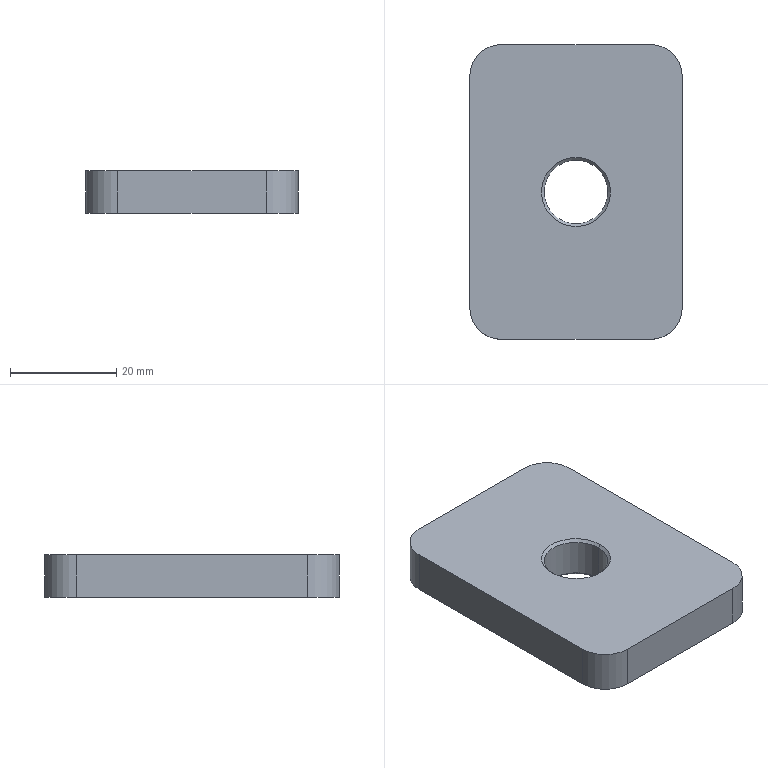Component | SolidWorks | 01-01Chassis-1_01-01-03ChassisWeldment3-1 | 1 solid | 16 faces | box 40 x 55.5 x 8 mm | volume 16598 mm3 | cylinder 6 | plane 6 | cone 4 | commonest cylinder face diameters 12 x6 | material Q235
STEP:
#1=COLOUR_RGB('',0.7922,0.8196,0.9333);
#2=FILL_AREA_STYLE_COLOUR('',#1);
#3=FILL_AREA_STYLE('',(#2));
#4=SURFACE_STYLE_FILL_AREA(#3);
#5=SURFACE_SIDE_STYLE('',(#4));
#6=SURFACE_STYLE_USAGE(.BOTH.,#5);
#7=PRESENTATION_STYLE_ASSIGNMENT((#6));
#8=CARTESIAN_POINT('',(11.575,-2.096,17.815));
#9=VERTEX_POINT('',#8);
#10=CARTESIAN_POINT('',(12.047,-2.096,17.815));
#11=VERTEX_POINT('',#10);
#12=CARTESIAN_POINT('',(11.811,-2.096,17.815));
#13=DIRECTION('',(0.,-0.,1.));
#14=DIRECTION('',(-1.,0.,0.));
#15=AXIS2_PLACEMENT_3D('',#12,#13,#14);
#16=CIRCLE('',#15,0.2362);
#17=EDGE_CURVE('',#9,#11,#16,.T.);
#18=ORIENTED_EDGE('',*,*,#17,.F.);
#19=CARTESIAN_POINT('',(11.555,-2.096,17.835));
#20=VERTEX_POINT('',#19);
#21=CARTESIAN_POINT('',(11.575,-2.096,17.815));
#22=DIRECTION('',(-0.7071,-0.,0.7071));
#23=VECTOR('',#22,39.37);
#24=LINE('',#21,#23);
#25=EDGE_CURVE('',#9,#20,#24,.T.);
#26=ORIENTED_EDGE('',*,*,#25,.T.);
#27=CARTESIAN_POINT('',(12.067,-2.096,17.835));
#28=VERTEX_POINT('',#27);
#29=CARTESIAN_POINT('',(11.811,-2.096,17.835));
#30=DIRECTION('',(-0.,0.,-1.));
#31=DIRECTION('',(-1.,0.,0.));
#32=AXIS2_PLACEMENT_3D('',#29,#30,#31);
#33=CIRCLE('',#32,0.2559);
#34=EDGE_CURVE('',#28,#20,#33,.T.);
#35=ORIENTED_EDGE('',*,*,#34,.F.);
#36=CARTESIAN_POINT('',(12.047,-2.096,17.815));
#37=DIRECTION('',(0.7071,-0.,0.7071));
#38=VECTOR('',#37,39.37);
#39=LINE('',#36,#38);
#40=EDGE_CURVE('',#11,#28,#39,.T.);
#41=ORIENTED_EDGE('',*,*,#40,.F.);
#42=EDGE_LOOP('',(#18,#26,#35,#41));
#43=FACE_OUTER_BOUND('',#42,.T.);
#44=CARTESIAN_POINT('',(11.811,-2.096,17.815));
#45=DIRECTION('',(0.,-0.,1.));
#46=DIRECTION('',(1.,0.,0.));
#47=AXIS2_PLACEMENT_3D('',#44,#45,#46);
#48=CONICAL_SURFACE('',#47,0.2362,0.7854);
#49=ADVANCED_FACE('',(#43),#48,.F.);
#50=CARTESIAN_POINT('',(12.047,-2.096,17.539));
#51=VERTEX_POINT('',#50);
#52=CARTESIAN_POINT('',(11.575,-2.096,17.539));
#53=VERTEX_POINT('',#52);
#54=CARTESIAN_POINT('',(11.811,-2.096,17.539));
#55=DIRECTION('',(-0.,0.,-1.));
#56=DIRECTION('',(-1.,0.,0.));
#57=AXIS2_PLACEMENT_3D('',#54,#55,#56);
#58=CIRCLE('',#57,0.2362);
#59=EDGE_CURVE('',#51,#53,#58,.T.);
#60=ORIENTED_EDGE('',*,*,#59,.F.);
#61=CARTESIAN_POINT('',(12.067,-2.096,17.52));
#62=VERTEX_POINT('',#61);
#63=CARTESIAN_POINT('',(12.047,-2.096,17.539));
#64=DIRECTION('',(0.7071,0.,-0.7071));
#65=VECTOR('',#64,39.37);
#66=LINE('',#63,#65);
#67=EDGE_CURVE('',#51,#62,#66,.T.);
#68=ORIENTED_EDGE('',*,*,#67,.T.);
#69=CARTESIAN_POINT('',(11.555,-2.096,17.52));
#70=VERTEX_POINT('',#69);
#71=CARTESIAN_POINT('',(11.811,-2.096,17.52));
#72=DIRECTION('',(0.,-0.,1.));
#73=DIRECTION('',(-1.,0.,0.));
#74=AXIS2_PLACEMENT_3D('',#71,#72,#73);
#75=CIRCLE('',#74,0.2559);
#76=EDGE_CURVE('',#70,#62,#75,.T.);
#77=ORIENTED_EDGE('',*,*,#76,.F.);
#78=CARTESIAN_POINT('',(11.575,-2.096,17.539));
#79=DIRECTION('',(-0.7071,0.,-0.7071));
#80=VECTOR('',#79,39.37);
#81=LINE('',#78,#80);
#82=EDGE_CURVE('',#53,#70,#81,.T.);
#83=ORIENTED_EDGE('',*,*,#82,.F.);
#84=EDGE_LOOP('',(#60,#68,#77,#83));
#85=FACE_OUTER_BOUND('',#84,.T.);
#86=CARTESIAN_POINT('',(11.811,-2.096,17.539));
#87=DIRECTION('',(-0.,0.,-1.));
#88=DIRECTION('',(-1.,0.,0.));
#89=AXIS2_PLACEMENT_3D('',#86,#87,#88);
#90=CONICAL_SURFACE('',#89,0.2362,0.7854);
#91=ADVANCED_FACE('',(#85),#90,.F.);
#92=ORIENTED_EDGE('',*,*,#59,.T.);
#93=CARTESIAN_POINT('',(11.575,-2.096,17.835));
#94=DIRECTION('',(0.,-0.,1.));
#95=VECTOR('',#94,39.37);
#96=LINE('',#93,#95);
#97=EDGE_CURVE('',#53,#9,#96,.T.);
#98=ORIENTED_EDGE('',*,*,#97,.T.);
#99=ORIENTED_EDGE('',*,*,#17,.T.);
#100=CARTESIAN_POINT('',(12.047,-2.096,17.835));
#101=DIRECTION('',(0.,-0.,1.));
#102=VECTOR('',#101,39.37);
#103=LINE('',#100,#102);
#104=EDGE_CURVE('',#51,#11,#103,.T.);
#105=ORIENTED_EDGE('',*,*,#104,.F.);
#106=EDGE_LOOP('',(#92,#98,#99,#105));
#107=FACE_OUTER_BOUND('',#106,.T.);
#108=CARTESIAN_POINT('',(11.811,-2.096,17.835));
#109=DIRECTION('',(0.,-0.,1.));
#110=DIRECTION('',(1.,0.,0.));
#111=AXIS2_PLACEMENT_3D('',#108,#109,#110);
#112=CYLINDRICAL_SURFACE('',#111,0.2362);
#113=ADVANCED_FACE('',(#107),#112,.F.);
#114=ORIENTED_EDGE('',*,*,#34,.T.);
#115=CARTESIAN_POINT('',(11.811,-2.096,17.835));
#116=DIRECTION('',(-0.,0.,-1.));
#117=DIRECTION('',(-1.,0.,0.));
#118=AXIS2_PLACEMENT_3D('',#115,#116,#117);
#119=CIRCLE('',#118,0.2559);
#120=EDGE_CURVE('',#20,#28,#119,.T.);
#121=ORIENTED_EDGE('',*,*,#120,.T.);
#122=EDGE_LOOP('',(#114,#121));
#123=FACE_BOUND('',#122,.T.);
#124=CARTESIAN_POINT('',(12.362,-1.004,17.835));
#125=VERTEX_POINT('',#124);
#126=CARTESIAN_POINT('',(12.598,-1.24,17.835));
#127=VERTEX_POINT('',#126);
#128=CARTESIAN_POINT('',(12.362,-1.24,17.835));
#129=DIRECTION('',(-0.,0.,-1.));
#130=DIRECTION('',(-1.,0.,0.));
#131=AXIS2_PLACEMENT_3D('',#128,#129,#130);
#132=CIRCLE('',#131,0.2362);
#133=EDGE_CURVE('',#125,#127,#132,.T.);
#134=ORIENTED_EDGE('',*,*,#133,.F.);
#135=CARTESIAN_POINT('',(11.26,-1.004,17.835));
#136=VERTEX_POINT('',#135);
#137=CARTESIAN_POINT('',(11.26,-1.004,17.835));
#138=DIRECTION('',(1.,-0.,-0.));
#139=VECTOR('',#138,39.37);
#140=LINE('',#137,#139);
#141=EDGE_CURVE('',#136,#125,#140,.T.);
#142=ORIENTED_EDGE('',*,*,#141,.F.);
#143=CARTESIAN_POINT('',(11.024,-1.24,17.835));
#144=VERTEX_POINT('',#143);
#145=CARTESIAN_POINT('',(11.26,-1.24,17.835));
#146=DIRECTION('',(-0.,0.,-1.));
#147=DIRECTION('',(1.,0.,0.));
#148=AXIS2_PLACEMENT_3D('',#145,#146,#147);
#149=CIRCLE('',#148,0.2362);
#150=EDGE_CURVE('',#144,#136,#149,.T.);
#151=ORIENTED_EDGE('',*,*,#150,.F.);
#152=CARTESIAN_POINT('',(11.024,-2.953,17.835));
#153=VERTEX_POINT('',#152);
#154=CARTESIAN_POINT('',(11.024,-1.24,17.835));
#155=DIRECTION('',(0.,1.,0.));
#156=VECTOR('',#155,39.37);
#157=LINE('',#154,#156);
#158=EDGE_CURVE('',#153,#144,#157,.T.);
#159=ORIENTED_EDGE('',*,*,#158,.F.);
#160=CARTESIAN_POINT('',(11.26,-3.189,17.835));
#161=VERTEX_POINT('',#160);
#162=CARTESIAN_POINT('',(11.26,-2.953,17.835));
#163=DIRECTION('',(-0.,0.,-1.));
#164=DIRECTION('',(1.,0.,0.));
#165=AXIS2_PLACEMENT_3D('',#162,#163,#164);
#166=CIRCLE('',#165,0.2362);
#167=EDGE_CURVE('',#161,#153,#166,.T.);
#168=ORIENTED_EDGE('',*,*,#167,.F.);
#169=CARTESIAN_POINT('',(12.362,-3.189,17.835));
#170=VERTEX_POINT('',#169);
#171=CARTESIAN_POINT('',(11.26,-3.189,17.835));
#172=DIRECTION('',(-1.,0.,0.));
#173=VECTOR('',#172,39.37);
#174=LINE('',#171,#173);
#175=EDGE_CURVE('',#170,#161,#174,.T.);
#176=ORIENTED_EDGE('',*,*,#175,.F.);
#177=CARTESIAN_POINT('',(12.598,-2.953,17.835));
#178=VERTEX_POINT('',#177);
#179=CARTESIAN_POINT('',(12.362,-2.953,17.835));
#180=DIRECTION('',(-0.,0.,-1.));
#181=DIRECTION('',(1.,0.,0.));
#182=AXIS2_PLACEMENT_3D('',#179,#180,#181);
#183=CIRCLE('',#182,0.2362);
#184=EDGE_CURVE('',#178,#170,#183,.T.);
#185=ORIENTED_EDGE('',*,*,#184,.F.);
#186=CARTESIAN_POINT('',(12.598,-1.24,17.835));
#187=DIRECTION('',(-0.,-1.,-0.));
#188=VECTOR('',#187,39.37);
#189=LINE('',#186,#188);
#190=EDGE_CURVE('',#127,#178,#189,.T.);
#191=ORIENTED_EDGE('',*,*,#190,.F.);
#192=EDGE_LOOP('',(#134,#142,#151,#159,#168,#176,#185,#191));
#193=FACE_OUTER_BOUND('',#192,.T.);
#194=CARTESIAN_POINT('',(12.362,-1.24,17.835));
#195=DIRECTION('',(-0.,0.,-1.));
#196=DIRECTION('',(-1.,-0.,0.));
#197=AXIS2_PLACEMENT_3D('',#194,#195,#196);
#198=PLANE('',#197);
#199=ADVANCED_FACE('',(#123,#193),#198,.F.);
#200=CARTESIAN_POINT('',(12.362,-1.004,17.52));
#201=VERTEX_POINT('',#200);
#202=CARTESIAN_POINT('',(12.598,-1.24,17.52));
#203=VERTEX_POINT('',#202);
#204=CARTESIAN_POINT('',(12.362,-1.24,17.52));
#205=DIRECTION('',(-0.,0.,-1.));
#206=DIRECTION('',(-1.,0.,0.));
#207=AXIS2_PLACEMENT_3D('',#204,#205,#206);
#208=CIRCLE('',#207,0.2362);
#209=EDGE_CURVE('',#201,#203,#208,.T.);
#210=ORIENTED_EDGE('',*,*,#209,.F.);
#211=CARTESIAN_POINT('',(12.362,-1.004,17.835));
#212=DIRECTION('',(-0.,0.,-1.));
#213=VECTOR('',#212,39.37);
#214=LINE('',#211,#213);
#215=EDGE_CURVE('',#125,#201,#214,.T.);
#216=ORIENTED_EDGE('',*,*,#215,.F.);
#217=ORIENTED_EDGE('',*,*,#133,.T.);
#218=CARTESIAN_POINT('',(12.598,-1.24,17.835));
#219=DIRECTION('',(-0.,0.,-1.));
#220=VECTOR('',#219,39.37);
#221=LINE('',#218,#220);
#222=EDGE_CURVE('',#127,#203,#221,.T.);
#223=ORIENTED_EDGE('',*,*,#222,.T.);
#224=EDGE_LOOP('',(#210,#216,#217,#223));
#225=FACE_OUTER_BOUND('',#224,.T.);
#226=CARTESIAN_POINT('',(12.362,-1.24,17.835));
#227=DIRECTION('',(-0.,0.,-1.));
#228=DIRECTION('',(-1.,0.,0.));
#229=AXIS2_PLACEMENT_3D('',#226,#227,#228);
#230=CYLINDRICAL_SURFACE('',#229,0.2362);
#231=ADVANCED_FACE('',(#225),#230,.T.);
#232=CARTESIAN_POINT('',(11.26,-1.004,17.52));
#233=VERTEX_POINT('',#232);
#234=CARTESIAN_POINT('',(11.26,-1.004,17.52));
#235=DIRECTION('',(1.,-0.,-0.));
#236=VECTOR('',#235,39.37);
#237=LINE('',#234,#236);
#238=EDGE_CURVE('',#233,#201,#237,.T.);
#239=ORIENTED_EDGE('',*,*,#238,.F.);
#240=CARTESIAN_POINT('',(11.26,-1.004,17.835));
#241=DIRECTION('',(-0.,0.,-1.));
#242=VECTOR('',#241,39.37);
#243=LINE('',#240,#242);
#244=EDGE_CURVE('',#136,#233,#243,.T.);
#245=ORIENTED_EDGE('',*,*,#244,.F.);
#246=ORIENTED_EDGE('',*,*,#141,.T.);
#247=ORIENTED_EDGE('',*,*,#215,.T.);
#248=EDGE_LOOP('',(#239,#245,#246,#247));
#249=FACE_OUTER_BOUND('',#248,.T.);
#250=CARTESIAN_POINT('',(11.26,-1.004,17.835));
#251=DIRECTION('',(0.,1.,0.));
#252=DIRECTION('',(1.,-0.,-0.));
#253=AXIS2_PLACEMENT_3D('',#250,#251,#252);
#254=PLANE('',#253);
#255=ADVANCED_FACE('',(#249),#254,.T.);
#256=CARTESIAN_POINT('',(11.024,-1.24,17.52));
#257=VERTEX_POINT('',#256);
#258=CARTESIAN_POINT('',(11.26,-1.24,17.52));
#259=DIRECTION('',(-0.,0.,-1.));
#260=DIRECTION('',(1.,0.,0.));
#261=AXIS2_PLACEMENT_3D('',#258,#259,#260);
#262=CIRCLE('',#261,0.2362);
#263=EDGE_CURVE('',#257,#233,#262,.T.);
#264=ORIENTED_EDGE('',*,*,#263,.F.);
#265=CARTESIAN_POINT('',(11.024,-1.24,17.835));
#266=DIRECTION('',(-0.,0.,-1.));
#267=VECTOR('',#266,39.37);
#268=LINE('',#265,#267);
#269=EDGE_CURVE('',#144,#257,#268,.T.);
#270=ORIENTED_EDGE('',*,*,#269,.F.);
#271=ORIENTED_EDGE('',*,*,#150,.T.);
#272=ORIENTED_EDGE('',*,*,#244,.T.);
#273=EDGE_LOOP('',(#264,#270,#271,#272));
#274=FACE_OUTER_BOUND('',#273,.T.);
#275=CARTESIAN_POINT('',(11.26,-1.24,17.835));
#276=DIRECTION('',(-0.,0.,-1.));
#277=DIRECTION('',(-1.,0.,0.));
#278=AXIS2_PLACEMENT_3D('',#275,#276,#277);
#279=CYLINDRICAL_SURFACE('',#278,0.2362);
#280=ADVANCED_FACE('',(#274),#279,.T.);
#281=CARTESIAN_POINT('',(11.024,-2.953,17.52));
#282=VERTEX_POINT('',#281);
#283=CARTESIAN_POINT('',(11.024,-1.24,17.52));
#284=DIRECTION('',(0.,1.,0.));
#285=VECTOR('',#284,39.37);
#286=LINE('',#283,#285);
#287=EDGE_CURVE('',#282,#257,#286,.T.);
#288=ORIENTED_EDGE('',*,*,#287,.F.);
#289=CARTESIAN_POINT('',(11.024,-2.953,17.835));
#290=DIRECTION('',(-0.,0.,-1.));
#291=VECTOR('',#290,39.37);
#292=LINE('',#289,#291);
#293=EDGE_CURVE('',#153,#282,#292,.T.);
#294=ORIENTED_EDGE('',*,*,#293,.F.);
#295=ORIENTED_EDGE('',*,*,#158,.T.);
#296=ORIENTED_EDGE('',*,*,#269,.T.);
#297=EDGE_LOOP('',(#288,#294,#295,#296));
#298=FACE_OUTER_BOUND('',#297,.T.);
#299=CARTESIAN_POINT('',(11.024,-1.24,17.835));
#300=DIRECTION('',(-1.,-0.,0.));
#301=DIRECTION('',(0.,-0.,1.));
#302=AXIS2_PLACEMENT_3D('',#299,#300,#301);
#303=PLANE('',#302);
#304=ADVANCED_FACE('',(#298),#303,.T.);
#305=CARTESIAN_POINT('',(11.26,-3.189,17.52));
#306=VERTEX_POINT('',#305);
#307=CARTESIAN_POINT('',(11.26,-2.953,17.52));
#308=DIRECTION('',(-0.,0.,-1.));
#309=DIRECTION('',(1.,0.,0.));
#310=AXIS2_PLACEMENT_3D('',#307,#308,#309);
#311=CIRCLE('',#310,0.2362);
#312=EDGE_CURVE('',#306,#282,#311,.T.);
#313=ORIENTED_EDGE('',*,*,#312,.F.);
#314=CARTESIAN_POINT('',(11.26,-3.189,17.835));
#315=DIRECTION('',(-0.,0.,-1.));
#316=VECTOR('',#315,39.37);
#317=LINE('',#314,#316);
#318=EDGE_CURVE('',#161,#306,#317,.T.);
#319=ORIENTED_EDGE('',*,*,#318,.F.);
#320=ORIENTED_EDGE('',*,*,#167,.T.);
#321=ORIENTED_EDGE('',*,*,#293,.T.);
#322=EDGE_LOOP('',(#313,#319,#320,#321));
#323=FACE_OUTER_BOUND('',#322,.T.);
#324=CARTESIAN_POINT('',(11.26,-2.953,17.835));
#325=DIRECTION('',(-0.,0.,-1.));
#326=DIRECTION('',(-1.,0.,0.));
#327=AXIS2_PLACEMENT_3D('',#324,#325,#326);
#328=CYLINDRICAL_SURFACE('',#327,0.2362);
#329=ADVANCED_FACE('',(#323),#328,.T.);
#330=CARTESIAN_POINT('',(12.362,-3.189,17.52));
#331=VERTEX_POINT('',#330);
#332=CARTESIAN_POINT('',(11.26,-3.189,17.52));
#333=DIRECTION('',(-1.,0.,0.));
#334=VECTOR('',#333,39.37);
#335=LINE('',#332,#334);
#336=EDGE_CURVE('',#331,#306,#335,.T.);
#337=ORIENTED_EDGE('',*,*,#336,.F.);
#338=CARTESIAN_POINT('',(12.362,-3.189,17.835));
#339=DIRECTION('',(-0.,0.,-1.));
#340=VECTOR('',#339,39.37);
#341=LINE('',#338,#340);
#342=EDGE_CURVE('',#170,#331,#341,.T.);
#343=ORIENTED_EDGE('',*,*,#342,.F.);
#344=ORIENTED_EDGE('',*,*,#175,.T.);
#345=ORIENTED_EDGE('',*,*,#318,.T.);
#346=EDGE_LOOP('',(#337,#343,#344,#345));
#347=FACE_OUTER_BOUND('',#346,.T.);
#348=CARTESIAN_POINT('',(11.26,-3.189,17.835));
#349=DIRECTION('',(-0.,-1.,-0.));
#350=DIRECTION('',(-1.,0.,0.));
#351=AXIS2_PLACEMENT_3D('',#348,#349,#350);
#352=PLANE('',#351);
#353=ADVANCED_FACE('',(#347),#352,.T.);
#354=CARTESIAN_POINT('',(12.598,-2.953,17.52));
#355=VERTEX_POINT('',#354);
#356=CARTESIAN_POINT('',(12.362,-2.953,17.52));
#357=DIRECTION('',(-0.,0.,-1.));
#358=DIRECTION('',(1.,0.,0.));
#359=AXIS2_PLACEMENT_3D('',#356,#357,#358);
#360=CIRCLE('',#359,0.2362);
#361=EDGE_CURVE('',#355,#331,#360,.T.);
#362=ORIENTED_EDGE('',*,*,#361,.F.);
#363=CARTESIAN_POINT('',(12.598,-2.953,17.835));
#364=DIRECTION('',(-0.,0.,-1.));
#365=VECTOR('',#364,39.37);
#366=LINE('',#363,#365);
#367=EDGE_CURVE('',#178,#355,#366,.T.);
#368=ORIENTED_EDGE('',*,*,#367,.F.);
#369=ORIENTED_EDGE('',*,*,#184,.T.);
#370=ORIENTED_EDGE('',*,*,#342,.T.);
#371=EDGE_LOOP('',(#362,#368,#369,#370));
#372=FACE_OUTER_BOUND('',#371,.T.);
#373=CARTESIAN_POINT('',(12.362,-2.953,17.835));
#374=DIRECTION('',(-0.,0.,-1.));
#375=DIRECTION('',(-1.,0.,0.));
#376=AXIS2_PLACEMENT_3D('',#373,#374,#375);
#377=CYLINDRICAL_SURFACE('',#376,0.2362);
#378=ADVANCED_FACE('',(#372),#377,.T.);
#379=CARTESIAN_POINT('',(12.598,-1.24,17.52));
#380=DIRECTION('',(-0.,-1.,-0.));
#381=VECTOR('',#380,39.37);
#382=LINE('',#379,#381);
#383=EDGE_CURVE('',#203,#355,#382,.T.);
#384=ORIENTED_EDGE('',*,*,#383,.F.);
#385=ORIENTED_EDGE('',*,*,#222,.F.);
#386=ORIENTED_EDGE('',*,*,#190,.T.);
#387=ORIENTED_EDGE('',*,*,#367,.T.);
#388=EDGE_LOOP('',(#384,#385,#386,#387));
#389=FACE_OUTER_BOUND('',#388,.T.);
#390=CARTESIAN_POINT('',(12.598,-1.24,17.835));
#391=DIRECTION('',(1.,-0.,-0.));
#392=DIRECTION('',(-0.,-1.,-0.));
#393=AXIS2_PLACEMENT_3D('',#390,#391,#392);
#394=PLANE('',#393);
#395=ADVANCED_FACE('',(#389),#394,.T.);
#396=ORIENTED_EDGE('',*,*,#76,.T.);
#397=CARTESIAN_POINT('',(11.811,-2.096,17.52));
#398=DIRECTION('',(0.,-0.,1.));
#399=DIRECTION('',(-1.,0.,0.));
#400=AXIS2_PLACEMENT_3D('',#397,#398,#399);
#401=CIRCLE('',#400,0.2559);
#402=EDGE_CURVE('',#62,#70,#401,.T.);
#403=ORIENTED_EDGE('',*,*,#402,.T.);
#404=EDGE_LOOP('',(#396,#403));
#405=FACE_BOUND('',#404,.T.);
#406=ORIENTED_EDGE('',*,*,#209,.T.);
#407=ORIENTED_EDGE('',*,*,#383,.T.);
#408=ORIENTED_EDGE('',*,*,#361,.T.);
#409=ORIENTED_EDGE('',*,*,#336,.T.);
#410=ORIENTED_EDGE('',*,*,#312,.T.);
#411=ORIENTED_EDGE('',*,*,#287,.T.);
#412=ORIENTED_EDGE('',*,*,#263,.T.);
#413=ORIENTED_EDGE('',*,*,#238,.T.);
#414=EDGE_LOOP('',(#406,#407,#408,#409,#410,#411,#412,#413));
#415=FACE_OUTER_BOUND('',#414,.T.);
#416=CARTESIAN_POINT('',(12.362,-1.24,17.52));
#417=DIRECTION('',(-0.,0.,-1.));
#418=DIRECTION('',(-1.,-0.,0.));
#419=AXIS2_PLACEMENT_3D('',#416,#417,#418);
#420=PLANE('',#419);
#421=ADVANCED_FACE('',(#405,#415),#420,.T.);
#422=ORIENTED_EDGE('',*,*,#97,.F.);
#423=CARTESIAN_POINT('',(11.811,-2.096,17.539));
#424=DIRECTION('',(-0.,0.,-1.));
#425=DIRECTION('',(-1.,0.,0.));
#426=AXIS2_PLACEMENT_3D('',#423,#424,#425);
#427=CIRCLE('',#426,0.2362);
#428=EDGE_CURVE('',#53,#51,#427,.T.);
#429=ORIENTED_EDGE('',*,*,#428,.T.);
#430=ORIENTED_EDGE('',*,*,#104,.T.);
#431=CARTESIAN_POINT('',(11.811,-2.096,17.815));
#432=DIRECTION('',(0.,-0.,1.));
#433=DIRECTION('',(-1.,0.,0.));
#434=AXIS2_PLACEMENT_3D('',#431,#432,#433);
#435=CIRCLE('',#434,0.2362);
#436=EDGE_CURVE('',#11,#9,#435,.T.);
#437=ORIENTED_EDGE('',*,*,#436,.T.);
#438=EDGE_LOOP('',(#422,#429,#430,#437));
#439=FACE_OUTER_BOUND('',#438,.T.);
#440=CARTESIAN_POINT('',(11.811,-2.096,17.835));
#441=DIRECTION('',(0.,-0.,1.));
#442=DIRECTION('',(1.,0.,0.));
#443=AXIS2_PLACEMENT_3D('',#440,#441,#442);
#444=CYLINDRICAL_SURFACE('',#443,0.2362);
#445=ADVANCED_FACE('',(#439),#444,.F.);
#446=ORIENTED_EDGE('',*,*,#67,.F.);
#447=ORIENTED_EDGE('',*,*,#428,.F.);
#448=ORIENTED_EDGE('',*,*,#82,.T.);
#449=ORIENTED_EDGE('',*,*,#402,.F.);
#450=EDGE_LOOP('',(#446,#447,#448,#449));
#451=FACE_OUTER_BOUND('',#450,.T.);
#452=CARTESIAN_POINT('',(11.811,-2.096,17.539));
#453=DIRECTION('',(-0.,0.,-1.));
#454=DIRECTION('',(-1.,0.,0.));
#455=AXIS2_PLACEMENT_3D('',#452,#453,#454);
#456=CONICAL_SURFACE('',#455,0.2362,0.7854);
#457=ADVANCED_FACE('',(#451),#456,.F.);
#458=ORIENTED_EDGE('',*,*,#25,.F.);
#459=ORIENTED_EDGE('',*,*,#436,.F.);
#460=ORIENTED_EDGE('',*,*,#40,.T.);
#461=ORIENTED_EDGE('',*,*,#120,.F.);
#462=EDGE_LOOP('',(#458,#459,#460,#461));
#463=FACE_OUTER_BOUND('',#462,.T.);
#464=CARTESIAN_POINT('',(11.811,-2.096,17.815));
#465=DIRECTION('',(0.,-0.,1.));
#466=DIRECTION('',(1.,0.,0.));
#467=AXIS2_PLACEMENT_3D('',#464,#465,#466);
#468=CONICAL_SURFACE('',#467,0.2362,0.7854);
#469=ADVANCED_FACE('',(#463),#468,.F.);
#470=CLOSED_SHELL('',(#49,#91,#113,#199,#231,#255,#280,#304,#329,#353,#378,#395,#421,#445,#457,#469));
#471=MANIFOLD_SOLID_BREP('',#470);
#472=STYLED_ITEM('',(#7),#471);
#473=PRESENTATION_LAYER_ASSIGNMENT('','',(#472));
#474=(LENGTH_UNIT()NAMED_UNIT(*)SI_UNIT($,.METRE.));
#475=LENGTH_MEASURE_WITH_UNIT(LENGTH_MEASURE(0.0254),#474);
#476=DIMENSIONAL_EXPONENTS(1.,0.,0.,0.,0.,0.,0.);
#477=(CONVERSION_BASED_UNIT('',#475)LENGTH_UNIT()NAMED_UNIT(#476));
#478=UNCERTAINTY_MEASURE_WITH_UNIT(LENGTH_MEASURE(0.00001),#477,'','');
#479=(NAMED_UNIT(*)PLANE_ANGLE_UNIT()SI_UNIT($,.RADIAN.));
#480=(NAMED_UNIT(*)SI_UNIT($,.STERADIAN.)SOLID_ANGLE_UNIT());
#481=(GEOMETRIC_REPRESENTATION_CONTEXT(3)GLOBAL_UNCERTAINTY_ASSIGNED_CONTEXT((#478))GLOBAL_UNIT_ASSIGNED_CONTEXT((#477,#479,#480))REPRESENTATION_CONTEXT('',''));
#482=MECHANICAL_DESIGN_GEOMETRIC_PRESENTATION_REPRESENTATION('',(#472),#481);
#483=CARTESIAN_POINT('',(0.,0.,0.));
#484=DIRECTION('',(0.,0.,1.));
#485=DIRECTION('',(1.,0.,0.));
#486=AXIS2_PLACEMENT_3D('',#483,#484,#485);
#487=(LENGTH_UNIT()NAMED_UNIT(*)SI_UNIT($,.METRE.));
#488=LENGTH_MEASURE_WITH_UNIT(LENGTH_MEASURE(0.0254),#487);
#489=DIMENSIONAL_EXPONENTS(1.,0.,0.,0.,0.,0.,0.);
#490=(CONVERSION_BASED_UNIT('',#488)LENGTH_UNIT()NAMED_UNIT(#489));
#491=UNCERTAINTY_MEASURE_WITH_UNIT(LENGTH_MEASURE(0.00001),#490,'','');
#492=(NAMED_UNIT(*)PLANE_ANGLE_UNIT()SI_UNIT($,.RADIAN.));
#493=(NAMED_UNIT(*)SI_UNIT($,.STERADIAN.)SOLID_ANGLE_UNIT());
#494=(GEOMETRIC_REPRESENTATION_CONTEXT(3)GLOBAL_UNCERTAINTY_ASSIGNED_CONTEXT((#491))GLOBAL_UNIT_ASSIGNED_CONTEXT((#490,#492,#493))REPRESENTATION_CONTEXT('',''));
#495=ADVANCED_BREP_SHAPE_REPRESENTATION('',(#471,#486),#494);